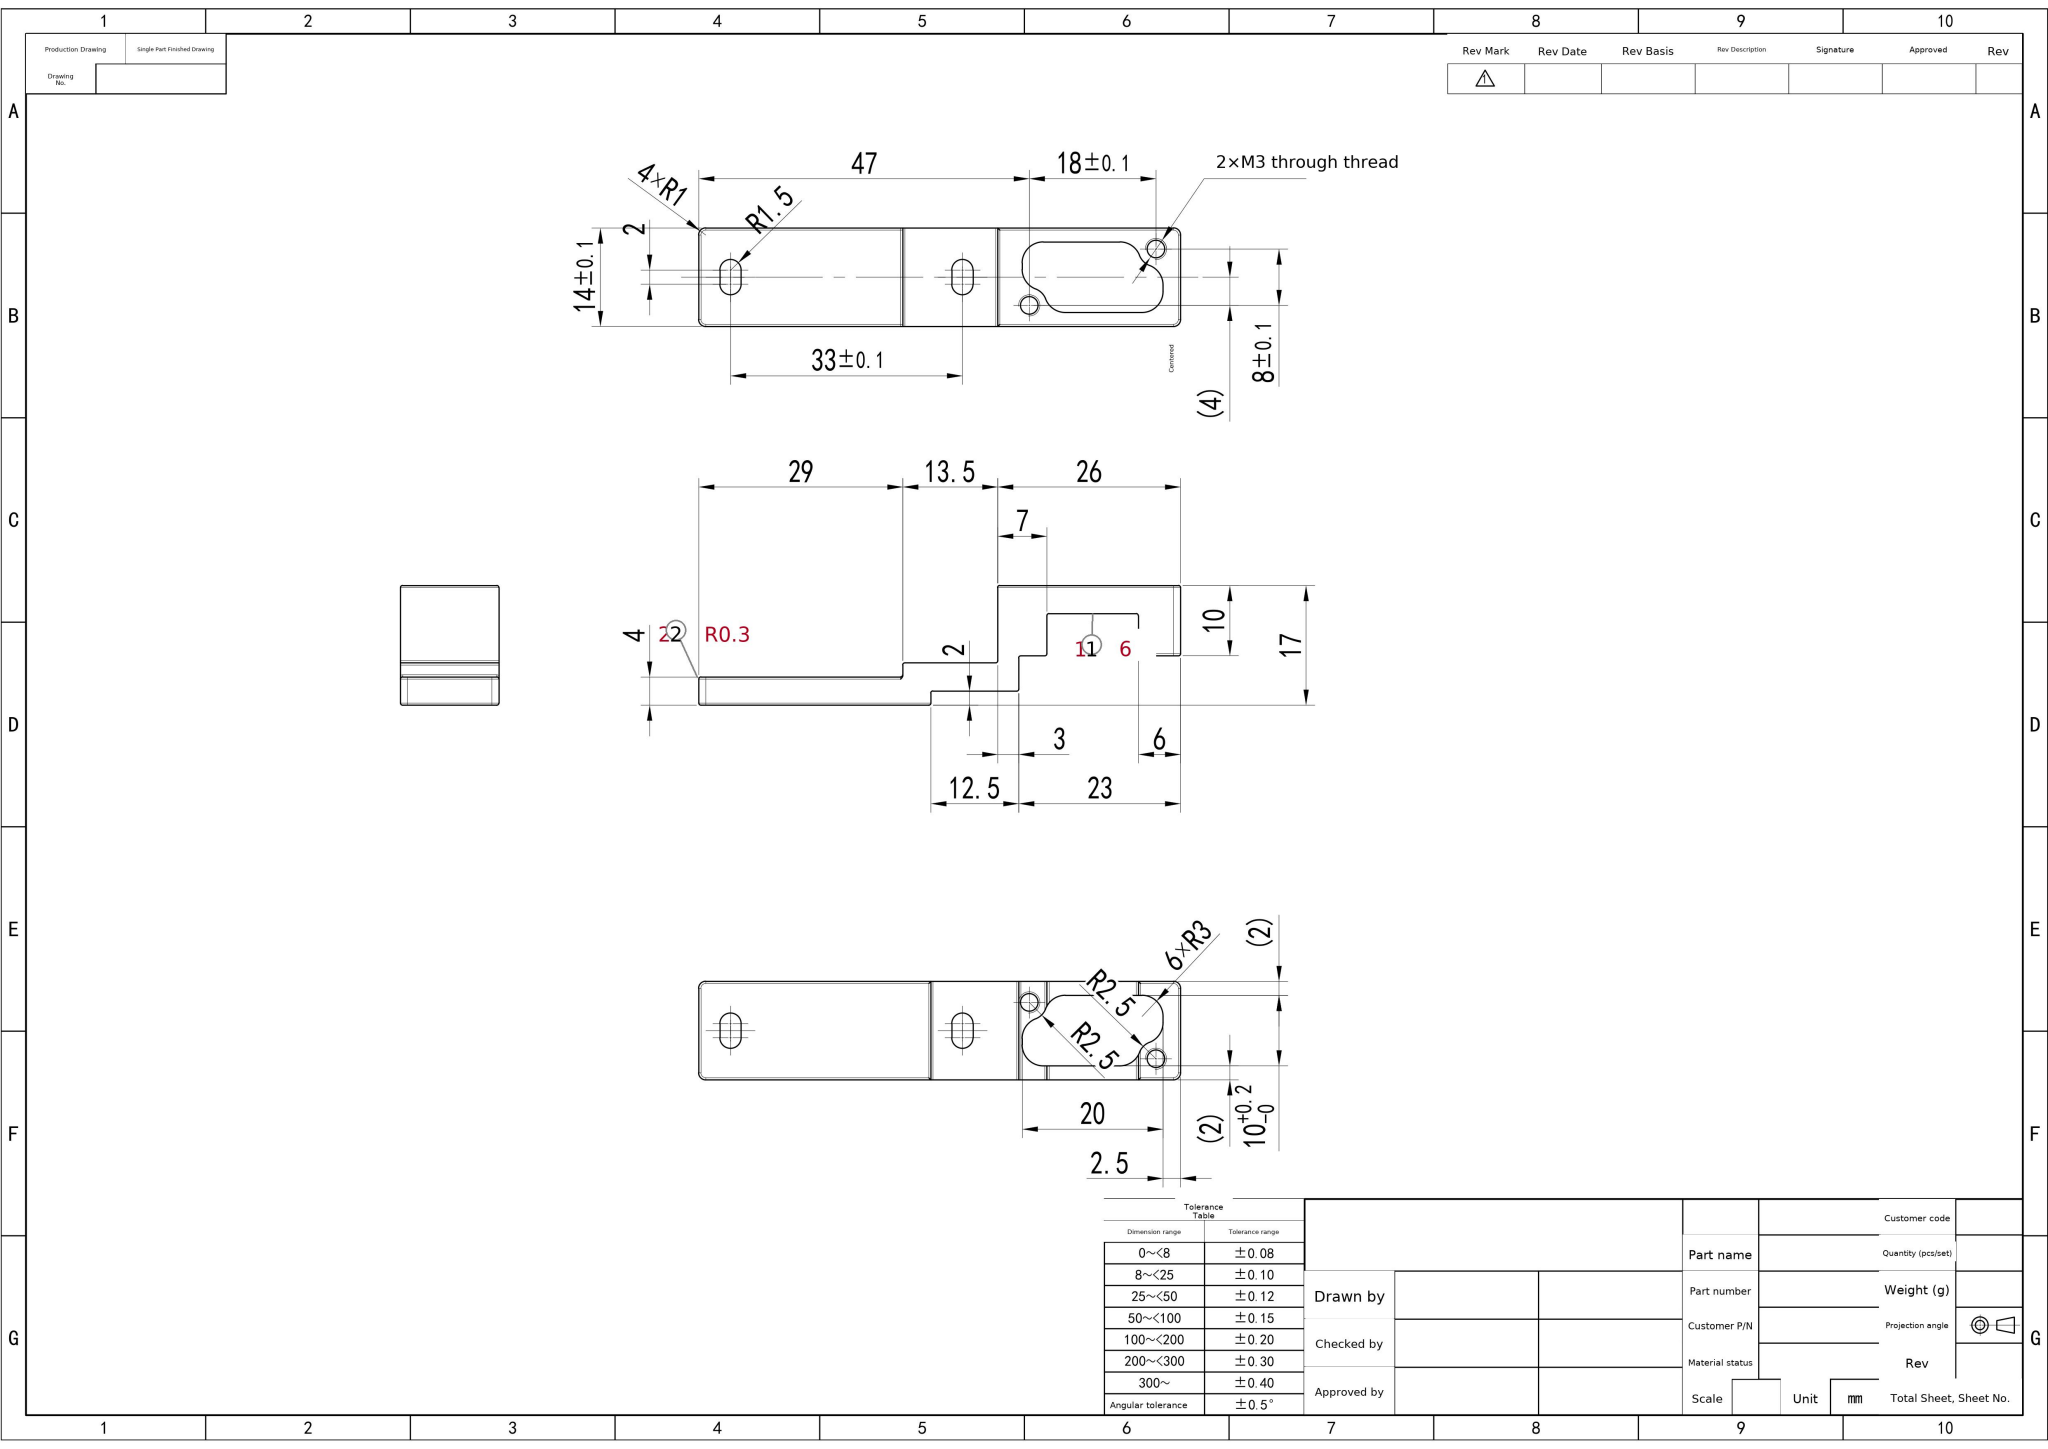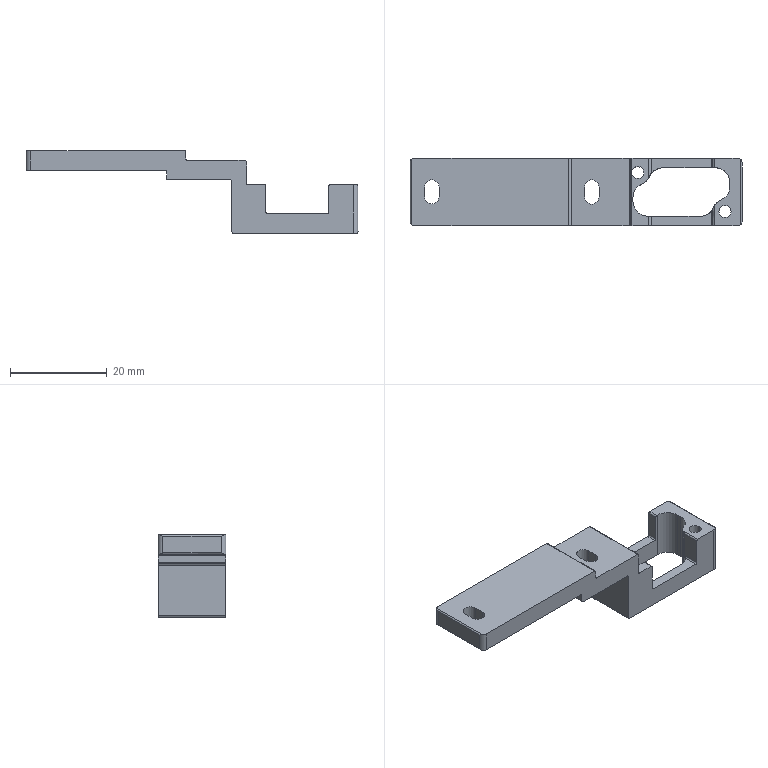Part | SolidWorks | mm | 1 solid | 69 faces | box 68.5 x 14 x 17 mm | volume 4111 mm3 | cylinder 38 | plane 29 | spline 2 | commonest cylinder face diameters 0.6 x18 6 x6 2.5 x4 3 x4 2 x4 5 x2